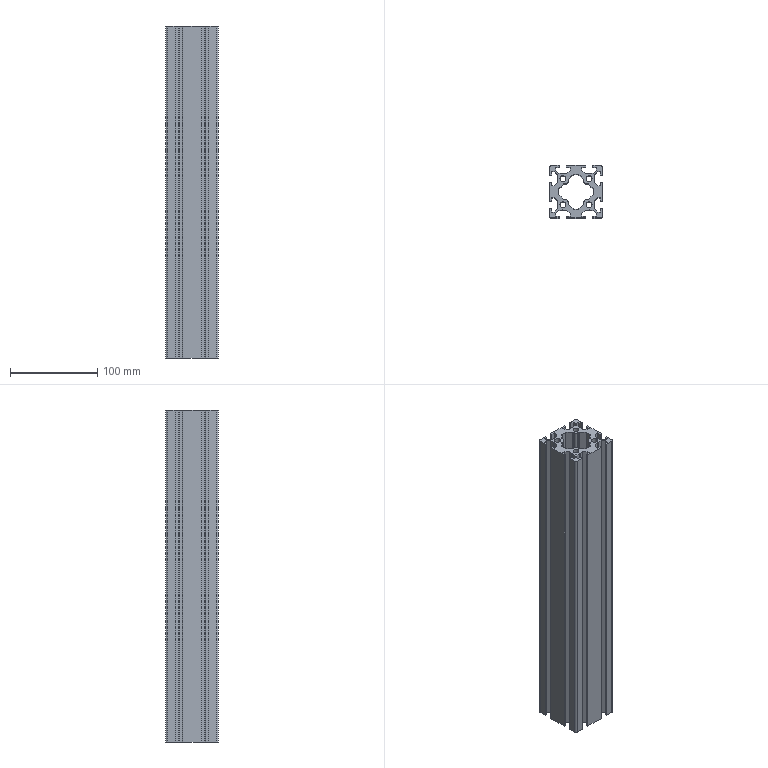Component | SolidWorks | E000-HFSG6_6060_380-2 | 1 solid | 178 faces | box 60 x 60 x 380 mm | volume 581098 mm3 | plane 130 | cylinder 48 | commonest cylinder face diameters 0.6 x16 2 x16 6.8 x8 4 x4 6 x4
build123d program:
from build123d import *

# Parameters (mm, degrees)
SKETCH1_R           = 3.4
BOSS_EXTRUDE1_DEPTH = 190


with BuildPart() as part:
    # Sketch1 → Boss-Extrude1 (new, symmetric)
    with BuildSketch(Plane.XY):
        with BuildLine():
            Line((-29.7, 19), (-28, 19))
            Line((-28, 19), (-28, 23.25))
            Line((-28, 23.25), (-24.664, 23.25))
            Line((-24.664, 23.25), (-21, 19.586))
            Line((-21, 19.586), (-21, 15.52))
            Line((-21, 15.52), (-20.7, 15))
            Line((-20.7, 15), (-21, 14.48))
            Line((-21, 14.48), (-21, 10.414))
            Line((-21, 10.414), (-24.664, 6.75))
            Line((-24.664, 6.75), (-28, 6.75))
            Line((-28, 6.75), (-28, 11))
            Line((-28, 11), (-29.7, 11))
            ThreePointArc((-29.7, 11), (-29.912, 10.912), (-30, 10.7))
            Line((-30, 10.7), (-30, -10.7))
            ThreePointArc((-30, -10.7), (-29.912, -10.912), (-29.7, -11))
            Line((-29.7, -11), (-28, -11))
            Line((-28, -11), (-28, -6.75))
            Line((-28, -6.75), (-24.664, -6.75))
            Line((-24.664, -6.75), (-21, -10.414))
            Line((-21, -10.414), (-21, -14.48))
            Line((-21, -14.48), (-20.7, -15))
            Line((-20.7, -15), (-21, -15.52))
            Line((-21, -15.52), (-21, -19.586))
            Line((-21, -19.586), (-24.664, -23.25))
            Line((-24.664, -23.25), (-28, -23.25))
            Line((-28, -23.25), (-28, -19))
            Line((-28, -19), (-29.7, -19))
            ThreePointArc((-29.7, -19), (-29.912, -19.088), (-30, -19.3))
            Line((-30, -19.3), (-30, -28))
            ThreePointArc((-30, -28), (-29.414, -29.414), (-28, -30))
            Line((-28, -30), (-19.3, -30))
            ThreePointArc((-19.3, -30), (-19.088, -29.912), (-19, -29.7))
            Line((-19, -29.7), (-19, -28))
            Line((-19, -28), (-23.25, -28))
            Line((-23.25, -28), (-23.25, -24.664))
            Line((-23.25, -24.664), (-19.586, -21))
            Line((-19.586, -21), (-15.52, -21))
            Line((-15.52, -21), (-15, -20.7))
            Line((-15, -20.7), (-14.48, -21))
            Line((-14.48, -21), (-10.414, -21))
            Line((-10.414, -21), (-6.75, -24.664))
            Line((-6.75, -24.664), (-6.75, -28))
            Line((-6.75, -28), (-11, -28))
            Line((-11, -28), (-11, -29.7))
            ThreePointArc((-11, -29.7), (-10.912, -29.912), (-10.7, -30))
            Line((-10.7, -30), (10.7, -30))
            ThreePointArc((10.7, -30), (10.912, -29.912), (11, -29.7))
            Line((11, -29.7), (11, -28))
            Line((11, -28), (6.75, -28))
            Line((6.75, -28), (6.75, -24.664))
            Line((6.75, -24.664), (10.414, -21))
            Line((10.414, -21), (14.48, -21))
            Line((14.48, -21), (15, -20.7))
            Line((15, -20.7), (15.52, -21))
            Line((15.52, -21), (19.586, -21))
            Line((19.586, -21), (23.25, -24.664))
            Line((23.25, -24.664), (23.25, -28))
            Line((23.25, -28), (19, -28))
            Line((19, -28), (19, -29.7))
            ThreePointArc((19, -29.7), (19.088, -29.912), (19.3, -30))
            Line((19.3, -30), (28, -30))
            ThreePointArc((28, -30), (29.414, -29.414), (30, -28))
            Line((30, -28), (30, -19.3))
            ThreePointArc((30, -19.3), (29.912, -19.088), (29.7, -19))
            Line((29.7, -19), (28, -19))
            Line((28, -19), (28, -23.25))
            Line((28, -23.25), (24.664, -23.25))
            Line((24.664, -23.25), (21, -19.586))
            Line((21, -19.586), (21, -15.52))
            Line((21, -15.52), (20.7, -15))
            Line((20.7, -15), (21, -14.48))
            Line((21, -14.48), (21, -10.414))
            Line((21, -10.414), (24.664, -6.75))
            Line((24.664, -6.75), (28, -6.75))
            Line((28, -6.75), (28, -11))
            Line((28, -11), (29.7, -11))
            ThreePointArc((29.7, -11), (29.912, -10.912), (30, -10.7))
            Line((30, -10.7), (30, 10.7))
            ThreePointArc((30, 10.7), (29.912, 10.912), (29.7, 11))
            Line((29.7, 11), (28, 11))
            Line((28, 11), (28, 6.75))
            Line((28, 6.75), (24.664, 6.75))
            Line((24.664, 6.75), (21, 10.414))
            Line((21, 10.414), (21, 14.48))
            Line((21, 14.48), (20.7, 15))
            Line((20.7, 15), (21, 15.52))
            Line((21, 15.52), (21, 19.586))
            Line((21, 19.586), (24.664, 23.25))
            Line((24.664, 23.25), (28, 23.25))
            Line((28, 23.25), (28, 19))
            Line((28, 19), (29.7, 19))
            ThreePointArc((29.7, 19), (29.912, 19.088), (30, 19.3))
            Line((30, 19.3), (30, 28))
            ThreePointArc((30, 28), (29.414, 29.414), (28, 30))
            Line((28, 30), (19.3, 30))
            ThreePointArc((19.3, 30), (19.088, 29.912), (19, 29.7))
            Line((19, 29.7), (19, 28))
            Line((19, 28), (23.25, 28))
            Line((23.25, 28), (23.25, 24.664))
            Line((23.25, 24.664), (19.586, 21))
            Line((19.586, 21), (15.52, 21))
            Line((15.52, 21), (15, 20.7))
            Line((15, 20.7), (14.48, 21))
            Line((14.48, 21), (10.414, 21))
            Line((10.414, 21), (6.75, 24.664))
            Line((6.75, 24.664), (6.75, 28))
            Line((6.75, 28), (11, 28))
            Line((11, 28), (11, 29.7))
            ThreePointArc((11, 29.7), (10.912, 29.912), (10.7, 30))
            Line((10.7, 30), (-10.7, 30))
            ThreePointArc((-10.7, 30), (-10.912, 29.912), (-11, 29.7))
            Line((-11, 29.7), (-11, 28))
            Line((-11, 28), (-6.75, 28))
            Line((-6.75, 28), (-6.75, 24.664))
            Line((-6.75, 24.664), (-10.414, 21))
            Line((-10.414, 21), (-14.48, 21))
            Line((-14.48, 21), (-15, 20.7))
            Line((-15, 20.7), (-15.52, 21))
            Line((-15.52, 21), (-19.586, 21))
            Line((-19.586, 21), (-23.25, 24.664))
            Line((-23.25, 24.664), (-23.25, 28))
            Line((-23.25, 28), (-19, 28))
            Line((-19, 28), (-19, 29.7))
            ThreePointArc((-19, 29.7), (-19.088, 29.912), (-19.3, 30))
            Line((-19.3, 30), (-28, 30))
            ThreePointArc((-28, 30), (-29.414, 29.414), (-30, 28))
            Line((-30, 28), (-30, 19.3))
            ThreePointArc((-30, 19.3), (-29.912, 19.088), (-29.7, 19))
        make_face()
        with Locations((15, 15)):
            Circle(SKETCH1_R, mode=Mode.SUBTRACT)
        with Locations((15, -15)):
            Circle(SKETCH1_R, mode=Mode.SUBTRACT)
        with Locations((-15, 15)):
            Circle(SKETCH1_R, mode=Mode.SUBTRACT)
        with Locations((-15, -15)):
            Circle(SKETCH1_R, mode=Mode.SUBTRACT)
        with BuildLine():
            Line((-19.707, -3.222), (-14.222, -8.707))
            ThreePointArc((-14.222, -8.707), (-13.897, -8.924), (-13.515, -9))
            Line((-13.515, -9), (-12, -9))
            ThreePointArc((-12, -9), (-9.879, -9.879), (-9, -12))
            Line((-9, -12), (-9, -13.515))
            ThreePointArc((-9, -13.515), (-8.924, -13.897), (-8.707, -14.222))
            Line((-8.707, -14.222), (-3.222, -19.707))
            ThreePointArc((-3.222, -19.707), (-2.897, -19.924), (-2.515, -20))
            Line((-2.515, -20), (2.515, -20))
            ThreePointArc((2.515, -20), (2.897, -19.924), (3.222, -19.707))
            Line((3.222, -19.707), (8.707, -14.222))
            ThreePointArc((8.707, -14.222), (8.924, -13.897), (9, -13.515))
            Line((9, -13.515), (9, -12))
            ThreePointArc((9, -12), (9.879, -9.879), (12, -9))
            Line((12, -9), (13.515, -9))
            ThreePointArc((13.515, -9), (13.897, -8.924), (14.222, -8.707))
            Line((14.222, -8.707), (19.707, -3.222))
            ThreePointArc((19.707, -3.222), (19.924, -2.897), (20, -2.515))
            Line((20, -2.515), (20, 2.515))
            ThreePointArc((20, 2.515), (19.924, 2.897), (19.707, 3.222))
            Line((19.707, 3.222), (14.222, 8.707))
            ThreePointArc((14.222, 8.707), (13.897, 8.924), (13.515, 9))
            Line((13.515, 9), (12, 9))
            ThreePointArc((12, 9), (9.879, 9.879), (9, 12))
            Line((9, 12), (9, 13.515))
            ThreePointArc((9, 13.515), (8.924, 13.897), (8.707, 14.222))
            Line((8.707, 14.222), (3.222, 19.707))
            ThreePointArc((3.222, 19.707), (2.897, 19.924), (2.515, 20))
            Line((2.515, 20), (-2.515, 20))
            ThreePointArc((-2.515, 20), (-2.897, 19.924), (-3.222, 19.707))
            Line((-3.222, 19.707), (-8.707, 14.222))
            ThreePointArc((-8.707, 14.222), (-8.924, 13.897), (-9, 13.515))
            Line((-9, 13.515), (-9, 12))
            ThreePointArc((-9, 12), (-9.879, 9.879), (-12, 9))
            Line((-12, 9), (-13.515, 9))
            ThreePointArc((-13.515, 9), (-13.897, 8.924), (-14.222, 8.707))
            Line((-14.222, 8.707), (-19.707, 3.222))
            ThreePointArc((-19.707, 3.222), (-19.924, 2.897), (-20, 2.515))
            Line((-20, 2.515), (-20, -2.515))
            ThreePointArc((-20, -2.515), (-19.924, -2.897), (-19.707, -3.222))
        make_face(mode=Mode.SUBTRACT)
    extrude(amount=BOSS_EXTRUDE1_DEPTH, both=True)


solid = part.part

# Placed as in the assembly
solid = solid.moved(Location((-220, 326, 0), (0, 0, 0)))